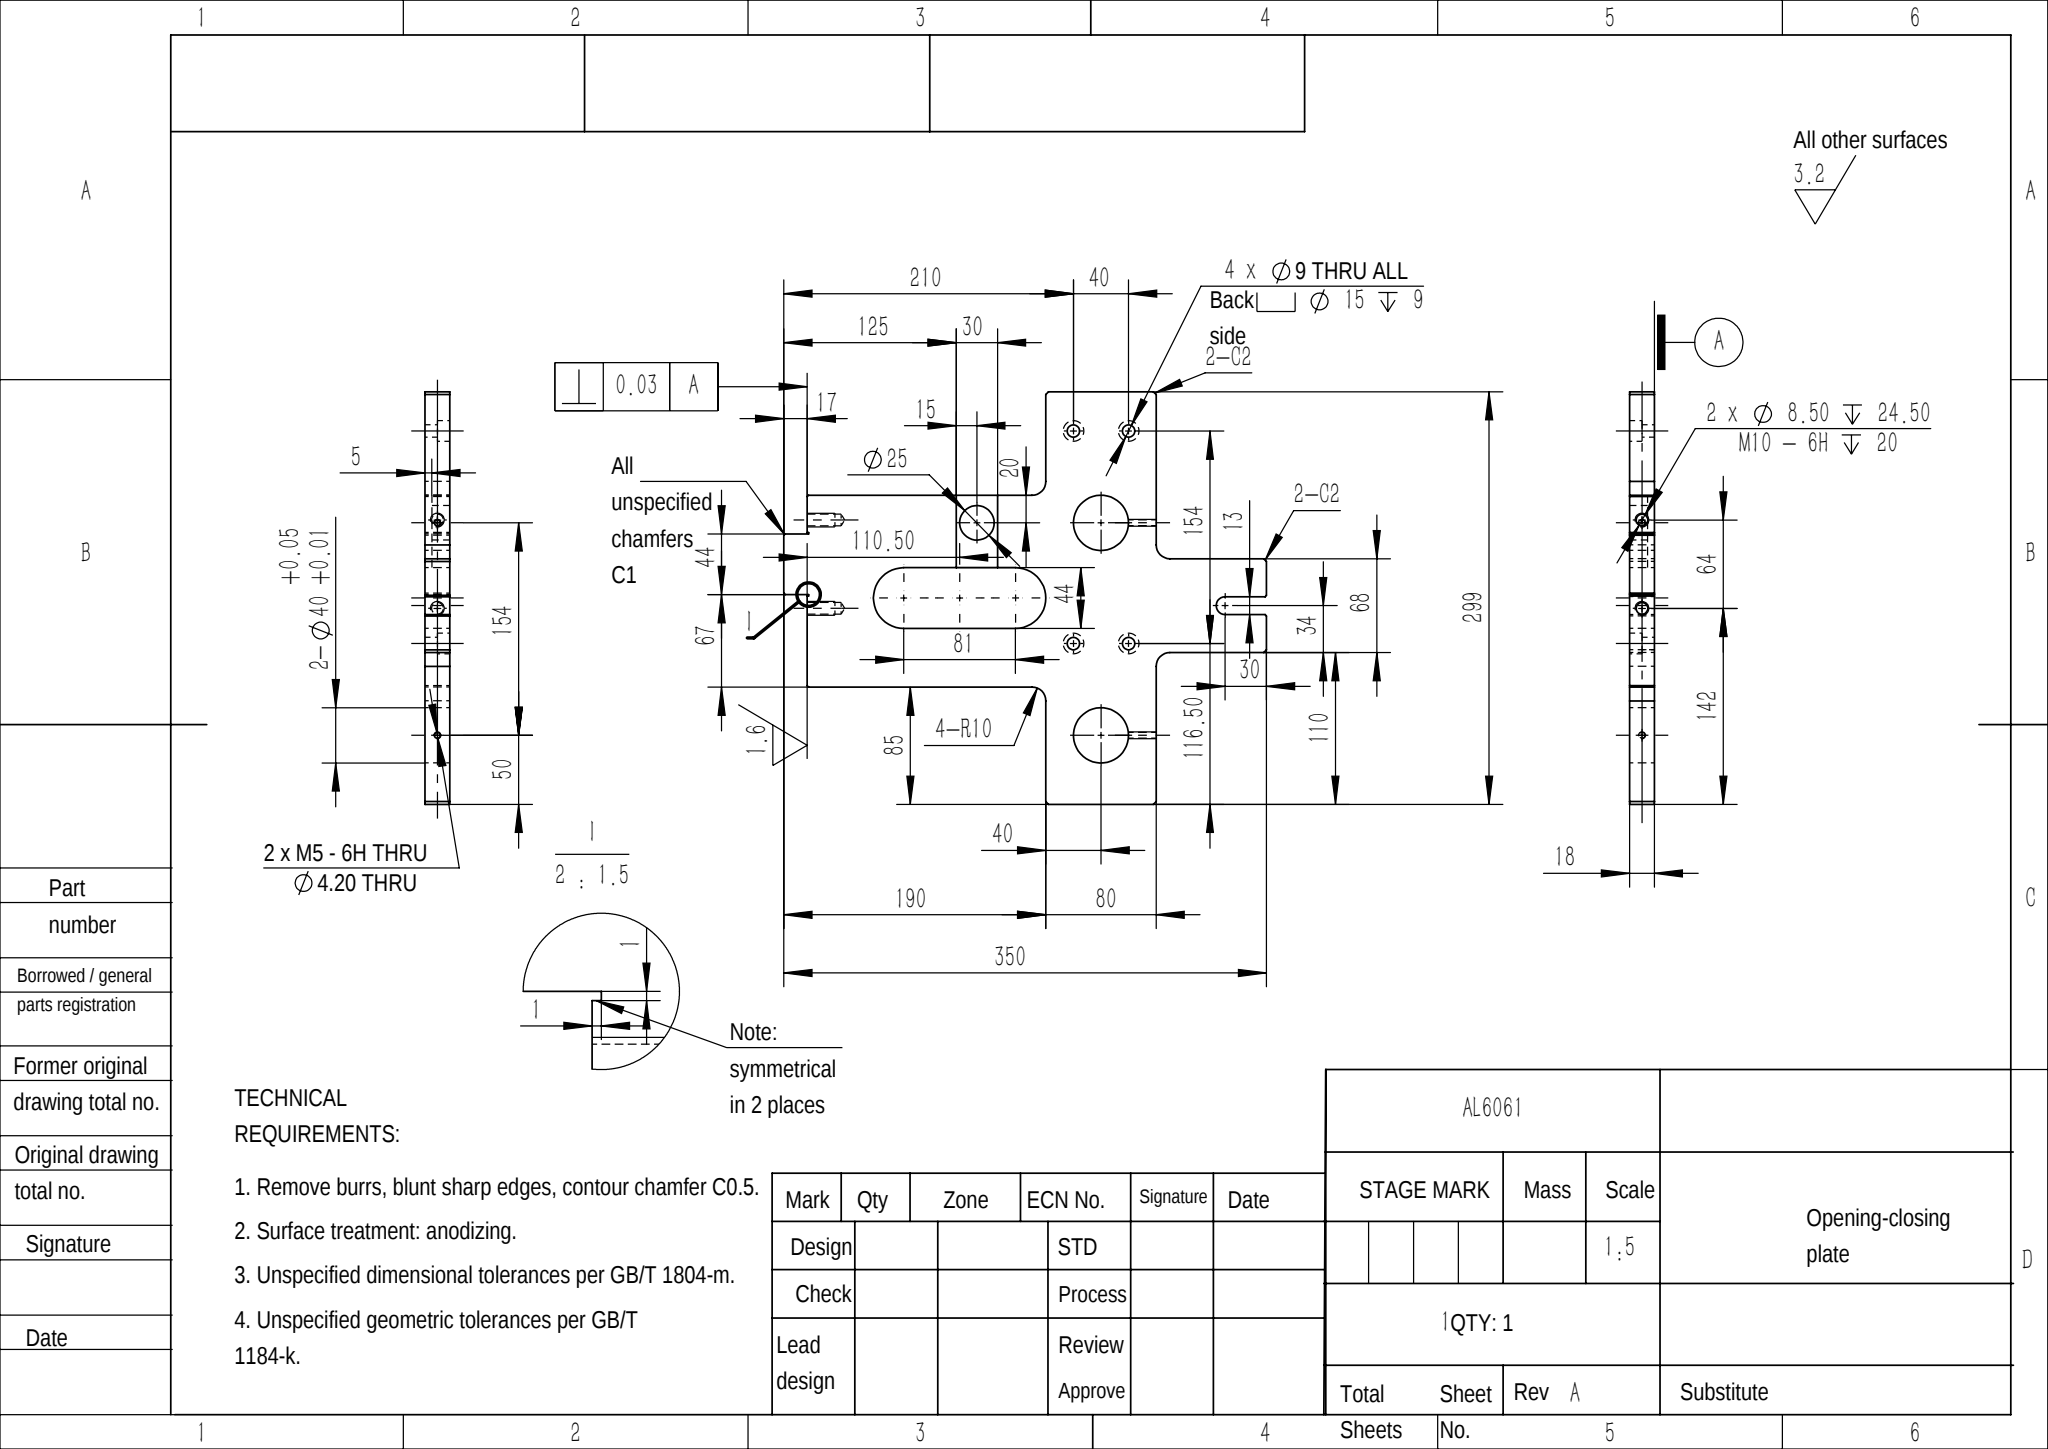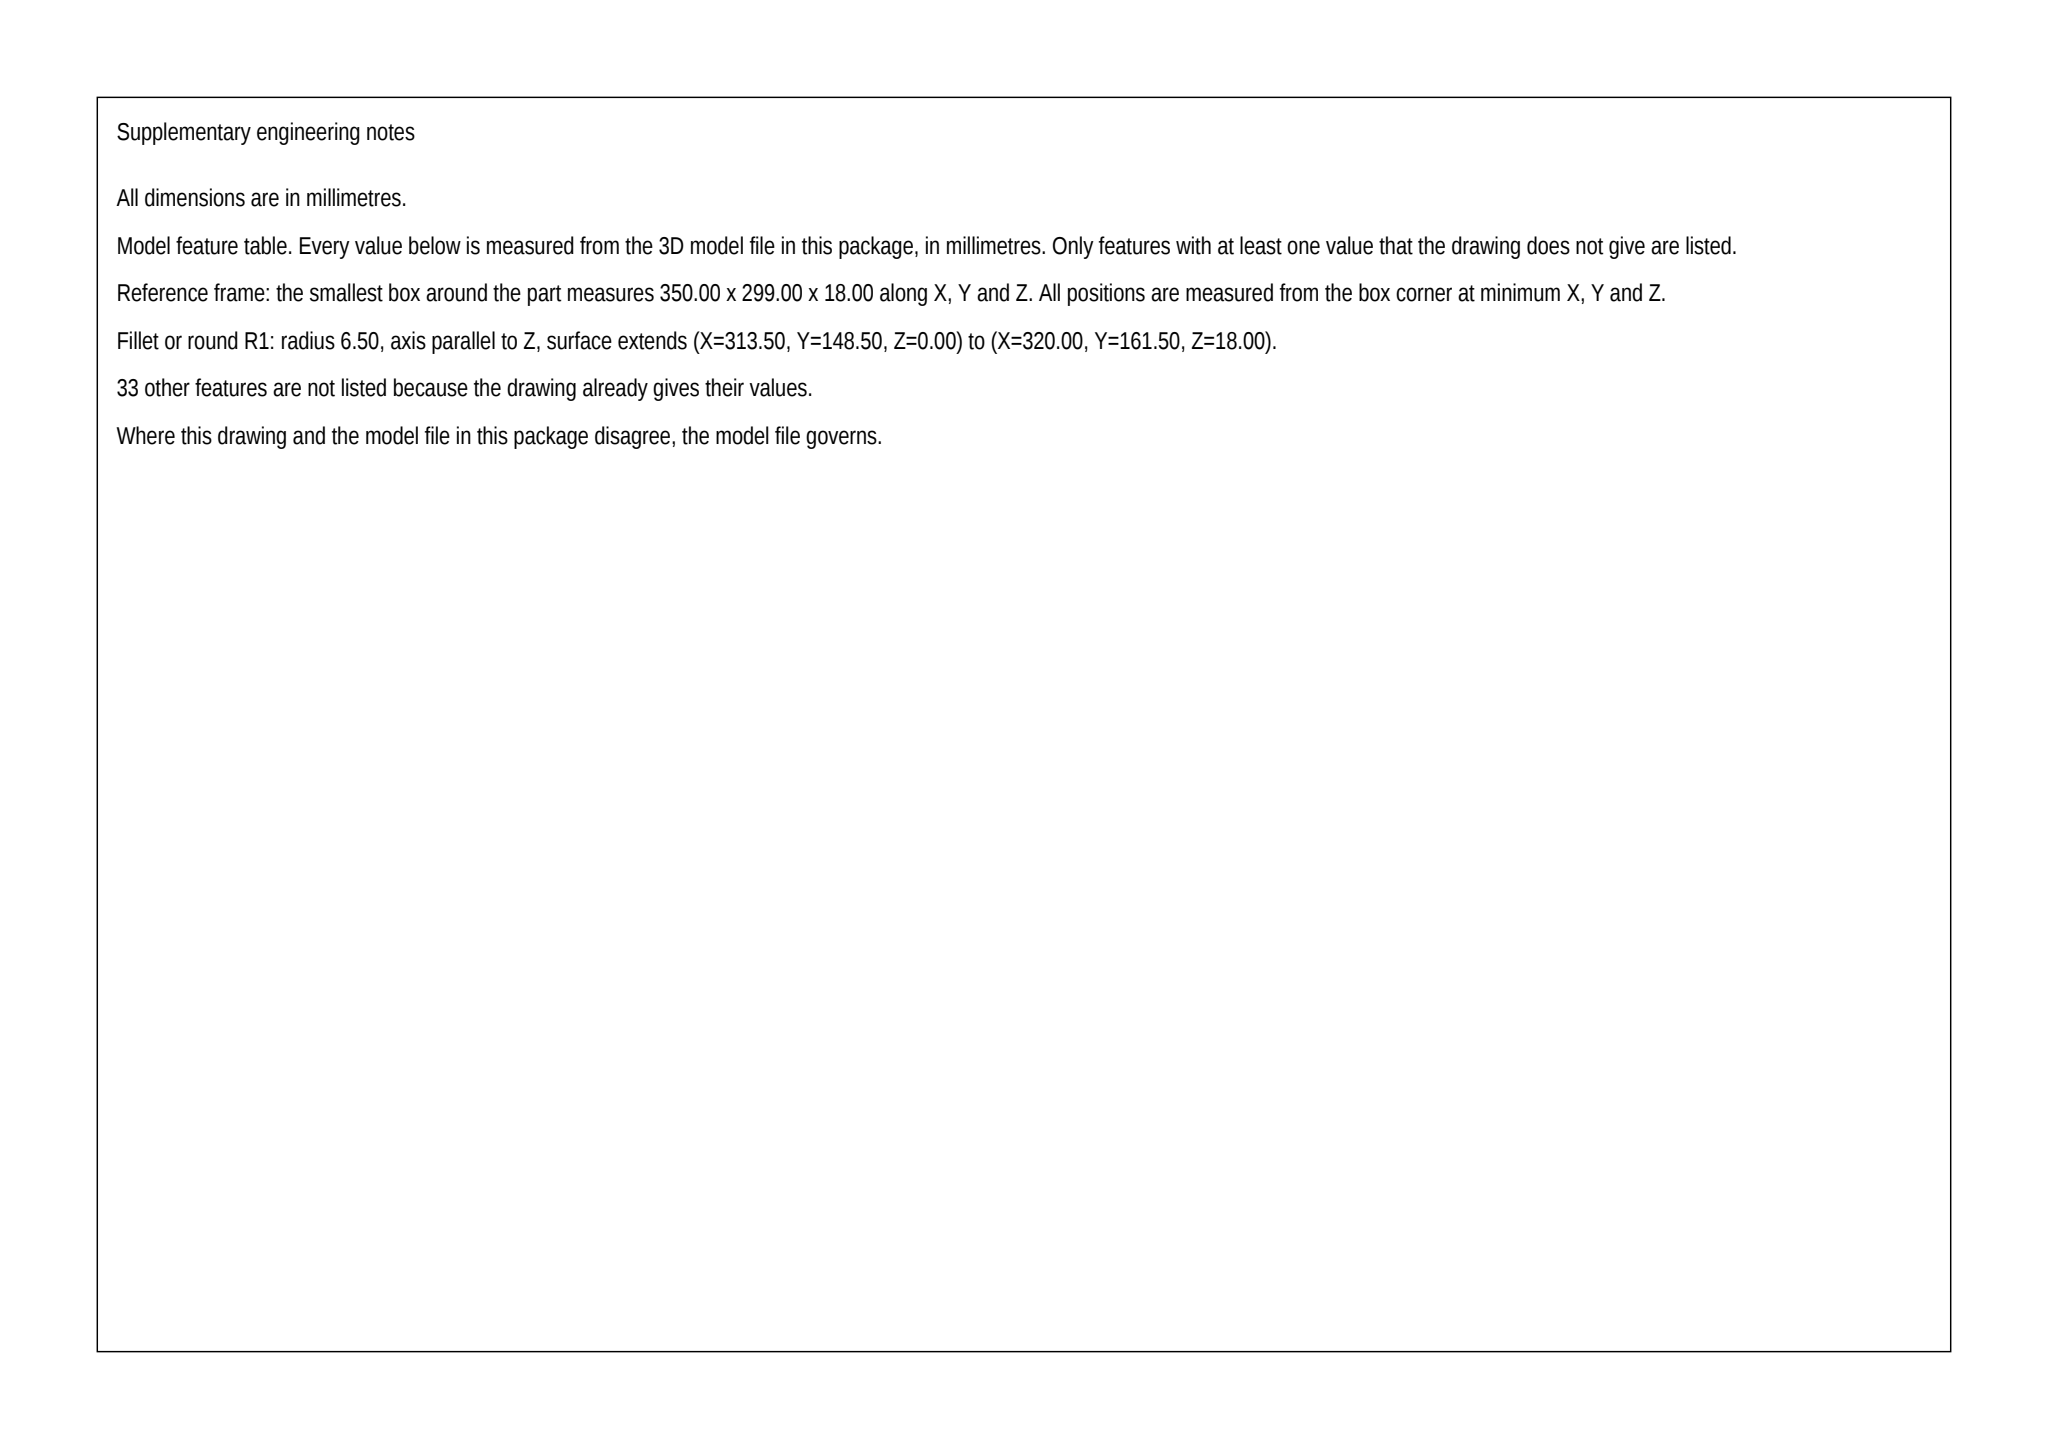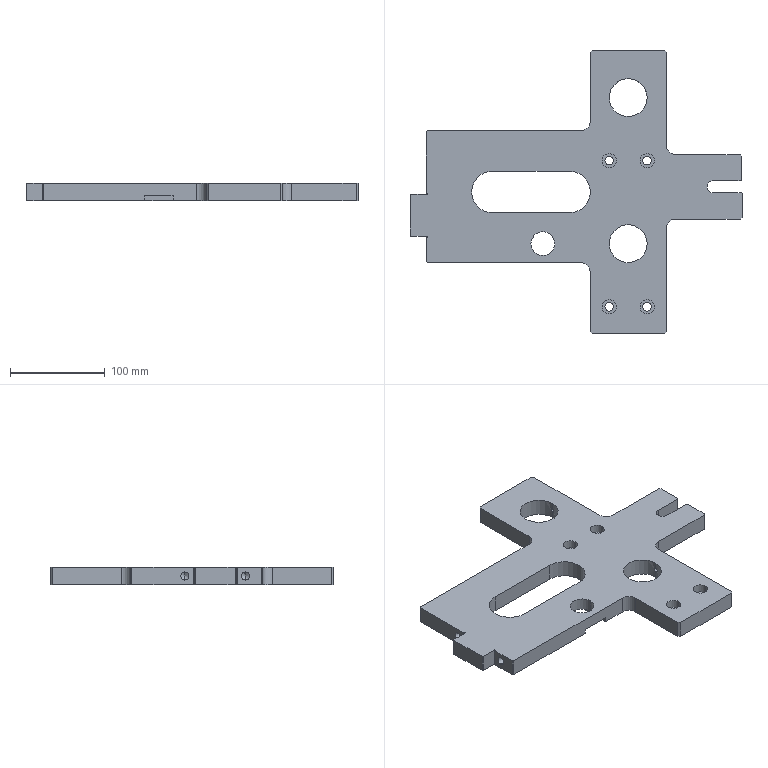Part | SolidWorks | mm | material AL6061 | 1 solid | 89 faces | box 350 x 299 x 18 mm | volume 804714 mm3 | plane 46 | cylinder 39 | cone 4 | commonest cylinder face diameters 15 x8 9 x8 4.2 x4 8.5 x4 40 x4 20 x4 44 x3 25 x2